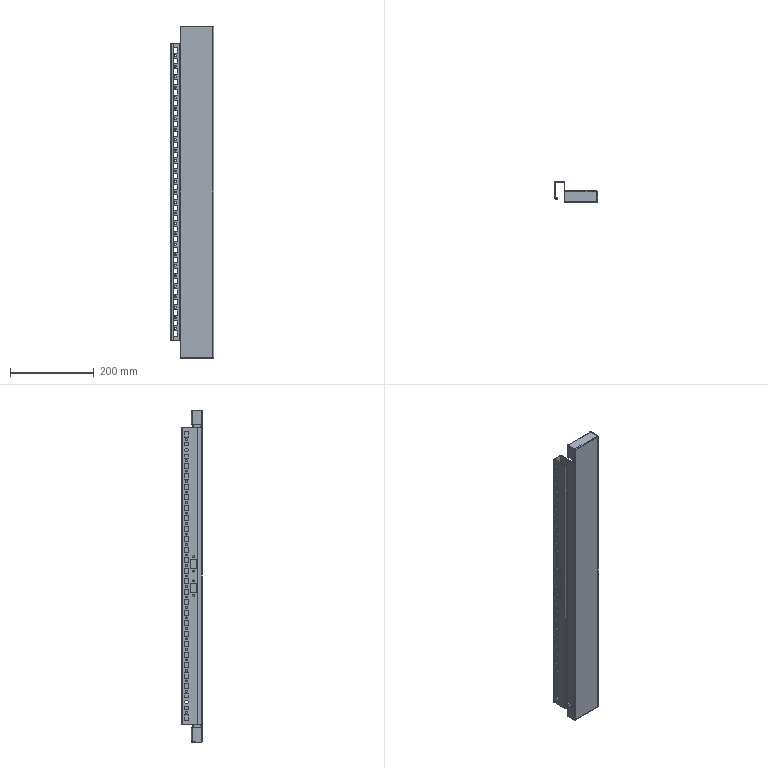Component | SolidWorks | LowerSealingPlateWeldingDrawingPG50-07-1_LowerCoverPlateWeldment1(PG50-07-101-1 | 1 solid | 532 faces | volume 336486 mm3 | plane 386 | cylinder 146 | commonest cylinder face diameters 4.6 x112 4.3 x12 0.3 x12 8.5 x4 3.4 x4 10 x2 | material AISI 1045 Steel, cold drawn